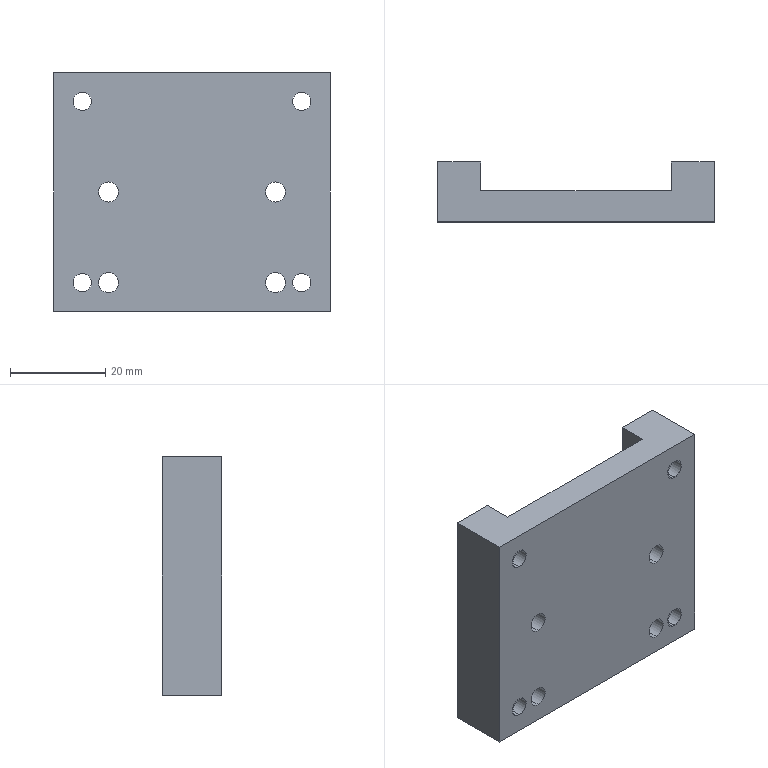Component | SolidWorks | PusherBlockSlideSeat-1 | 1 solid | 34 faces | box 58 x 12.5 x 50 mm | volume 23197 mm3 | cylinder 16 | plane 10 | cone 8 | commonest cylinder face diameters 4.2 x16
build123d program:
from build123d import *

# Parameters (mm, degrees)
SKETCH1_W             = 58
SKETCH1_H             = 50
BOSS_EXTRUDE1_DEPTH   = 12.5
SKETCH2_W             = 40
SKETCH2_H             = 78.188
CUT_EXTRUDE1_DEPTH    = 6
SKETCH6_W             = 20
SKETCH6_H             = 12.5
CUT_EXTRUDE2_DEPTH    = 12
BOSS_EXTRUDE2_DEPTH   = 12
M5_TAPPED_HOLE2_D     = 4.2
M5_TAPPED_HOLE2_DEPTH = 12.4
M5_TAPPED_HOLE2_TIP   = 1.262
M5_TAPPED_HOLE3_D     = 4.2
M5_TAPPED_HOLE3_DEPTH = 12.4
M5_TAPPED_HOLE3_TIP   = 1.262


with BuildPart() as part:
    # Sketch1 → Boss-Extrude1 (new body)
    with BuildSketch(Plane(origin=(0, 0, 0), x_dir=(1, 0, 0), z_dir=(0, 1, 0))):
        with Locations((-41.142, -16.579)):
            Rectangle(SKETCH1_W, SKETCH1_H)
    extrude(amount=BOSS_EXTRUDE1_DEPTH)

    # Sketch2 → Cut-Extrude1 (cut)
    with BuildSketch(Plane(origin=(0, 12.5, 0), x_dir=(1, 0, 0), z_dir=(0, 1, 0))):
        with Locations((-41.142, -23.387)):
            Rectangle(SKETCH2_W, SKETCH2_H)
    extrude(amount=-CUT_EXTRUDE1_DEPTH, mode=Mode.SUBTRACT)

    # Sketch6 → Cut-Extrude2 (cut)
    with BuildSketch(Plane.XY.offset(41.579)):
        with Locations((-22.142, 6.25)):
            Rectangle(SKETCH6_W, SKETCH6_H)
    extrude(amount=-CUT_EXTRUDE2_DEPTH, mode=Mode.SUBTRACT)

    # Sketch8 → Boss-Extrude2 (add)
    with BuildSketch(Plane.XY.offset(29.579)):
        Polygon((-32.142, 6.5), (-21.142, 6.5), (-21.142, 12.5), (-12.142, 12.5), (-12.142, 0), (-32.142, 0), align=None)
    extrude(amount=BOSS_EXTRUDE2_DEPTH)

    # M5 Tapped Hole2
    with Locations(Plane(origin=(0, 12.5, 0), x_dir=(-1, 0, 0), z_dir=(0, 1, 0))):
        with Locations((64.142, -2.421), (64.142, 35.579), (18.142, -2.421), (18.142, 35.579)):
            Hole(M5_TAPPED_HOLE2_D / 2, depth=M5_TAPPED_HOLE2_DEPTH)
            with Locations((0, 0, -(M5_TAPPED_HOLE2_DEPTH + M5_TAPPED_HOLE2_TIP / 2))):  # 118° drill point
                Cone(0, M5_TAPPED_HOLE2_D / 2, M5_TAPPED_HOLE2_TIP, mode=Mode.SUBTRACT)

    # M5 Tapped Hole3
    with Locations(Plane.XZ):
        with Locations((-23.642, -2.421), (-23.642, 16.579), (-58.642, 16.579), (-58.642, -2.421)):
            Hole(M5_TAPPED_HOLE3_D / 2, depth=M5_TAPPED_HOLE3_DEPTH)
            with Locations((0, 0, -(M5_TAPPED_HOLE3_DEPTH + M5_TAPPED_HOLE3_TIP / 2))):  # 118° drill point
                Cone(0, M5_TAPPED_HOLE3_D / 2, M5_TAPPED_HOLE3_TIP, mode=Mode.SUBTRACT)


solid = part.part

# Placed as in the assembly
solid = solid.moved(Location((34.227, -1.305, 60), (0, 0, 0)))
STEP:
#1=COLOUR_RGB('',0.7922,0.8196,0.9333);
#2=FILL_AREA_STYLE_COLOUR('',#1);
#3=FILL_AREA_STYLE('',(#2));
#4=SURFACE_STYLE_FILL_AREA(#3);
#5=SURFACE_SIDE_STYLE('',(#4));
#6=SURFACE_STYLE_USAGE(.BOTH.,#5);
#7=PRESENTATION_STYLE_ASSIGNMENT((#6));
#8=CARTESIAN_POINT('',(0.4167,0.2045,2.184));
#9=VERTEX_POINT('',#8);
#10=CARTESIAN_POINT('',(0.4167,0.2045,2.35));
#11=VERTEX_POINT('',#10);
#12=CARTESIAN_POINT('',(0.4167,0.2045,2.267));
#13=DIRECTION('',(0.,1.,0.));
#14=DIRECTION('',(0.,0.,1.));
#15=AXIS2_PLACEMENT_3D('',#12,#13,#14);
#16=CIRCLE('',#15,0.08268);
#17=EDGE_CURVE('',#9,#11,#16,.T.);
#18=ORIENTED_EDGE('',*,*,#17,.T.);
#19=CARTESIAN_POINT('',(0.4167,-0.05139,2.35));
#20=VERTEX_POINT('',#19);
#21=CARTESIAN_POINT('',(0.4167,-0.05139,2.35));
#22=DIRECTION('',(0.,-1.,0.));
#23=VECTOR('',#22,39.37);
#24=LINE('',#21,#23);
#25=EDGE_CURVE('',#11,#20,#24,.T.);
#26=ORIENTED_EDGE('',*,*,#25,.T.);
#27=CARTESIAN_POINT('',(0.4167,-0.05139,2.184));
#28=VERTEX_POINT('',#27);
#29=CARTESIAN_POINT('',(0.4167,-0.05139,2.267));
#30=DIRECTION('',(0.,-1.,0.));
#31=DIRECTION('',(0.,0.,-1.));
#32=AXIS2_PLACEMENT_3D('',#29,#30,#31);
#33=CIRCLE('',#32,0.08268);
#34=EDGE_CURVE('',#20,#28,#33,.T.);
#35=ORIENTED_EDGE('',*,*,#34,.T.);
#36=CARTESIAN_POINT('',(0.4167,-0.05139,2.184));
#37=DIRECTION('',(0.,-1.,0.));
#38=VECTOR('',#37,39.37);
#39=LINE('',#36,#38);
#40=EDGE_CURVE('',#9,#28,#39,.T.);
#41=ORIENTED_EDGE('',*,*,#40,.F.);
#42=EDGE_LOOP('',(#18,#26,#35,#41));
#43=FACE_OUTER_BOUND('',#42,.T.);
#44=CARTESIAN_POINT('',(0.4167,-0.05139,2.267));
#45=DIRECTION('',(0.,-1.,0.));
#46=DIRECTION('',(0.,0.,-1.));
#47=AXIS2_PLACEMENT_3D('',#44,#45,#46);
#48=CYLINDRICAL_SURFACE('',#47,0.08268);
#49=ADVANCED_FACE('',(#43),#48,.F.);
#50=CARTESIAN_POINT('',(0.4167,0.2045,2.932));
#51=VERTEX_POINT('',#50);
#52=CARTESIAN_POINT('',(0.4167,0.2045,3.098));
#53=VERTEX_POINT('',#52);
#54=CARTESIAN_POINT('',(0.4167,0.2045,3.015));
#55=DIRECTION('',(0.,1.,0.));
#56=DIRECTION('',(0.,0.,1.));
#57=AXIS2_PLACEMENT_3D('',#54,#55,#56);
#58=CIRCLE('',#57,0.08268);
#59=EDGE_CURVE('',#51,#53,#58,.T.);
#60=ORIENTED_EDGE('',*,*,#59,.T.);
#61=CARTESIAN_POINT('',(0.4167,-0.05139,3.098));
#62=VERTEX_POINT('',#61);
#63=CARTESIAN_POINT('',(0.4167,-0.05139,3.098));
#64=DIRECTION('',(0.,-1.,0.));
#65=VECTOR('',#64,39.37);
#66=LINE('',#63,#65);
#67=EDGE_CURVE('',#53,#62,#66,.T.);
#68=ORIENTED_EDGE('',*,*,#67,.T.);
#69=CARTESIAN_POINT('',(0.4167,-0.05139,2.932));
#70=VERTEX_POINT('',#69);
#71=CARTESIAN_POINT('',(0.4167,-0.05139,3.015));
#72=DIRECTION('',(0.,-1.,0.));
#73=DIRECTION('',(0.,0.,-1.));
#74=AXIS2_PLACEMENT_3D('',#71,#72,#73);
#75=CIRCLE('',#74,0.08268);
#76=EDGE_CURVE('',#62,#70,#75,.T.);
#77=ORIENTED_EDGE('',*,*,#76,.T.);
#78=CARTESIAN_POINT('',(0.4167,-0.05139,2.932));
#79=DIRECTION('',(0.,-1.,0.));
#80=VECTOR('',#79,39.37);
#81=LINE('',#78,#80);
#82=EDGE_CURVE('',#51,#70,#81,.T.);
#83=ORIENTED_EDGE('',*,*,#82,.F.);
#84=EDGE_LOOP('',(#60,#68,#77,#83));
#85=FACE_OUTER_BOUND('',#84,.T.);
#86=CARTESIAN_POINT('',(0.4167,-0.05139,3.015));
#87=DIRECTION('',(0.,-1.,0.));
#88=DIRECTION('',(0.,0.,-1.));
#89=AXIS2_PLACEMENT_3D('',#86,#87,#88);
#90=CYLINDRICAL_SURFACE('',#89,0.08268);
#91=ADVANCED_FACE('',(#85),#90,.F.);
#92=CARTESIAN_POINT('',(-0.9612,0.2045,2.932));
#93=VERTEX_POINT('',#92);
#94=CARTESIAN_POINT('',(-0.9612,0.2045,3.098));
#95=VERTEX_POINT('',#94);
#96=CARTESIAN_POINT('',(-0.9612,0.2045,3.015));
#97=DIRECTION('',(0.,1.,0.));
#98=DIRECTION('',(0.,0.,1.));
#99=AXIS2_PLACEMENT_3D('',#96,#97,#98);
#100=CIRCLE('',#99,0.08268);
#101=EDGE_CURVE('',#93,#95,#100,.T.);
#102=ORIENTED_EDGE('',*,*,#101,.T.);
#103=CARTESIAN_POINT('',(-0.9612,-0.05139,3.098));
#104=VERTEX_POINT('',#103);
#105=CARTESIAN_POINT('',(-0.9612,-0.05139,3.098));
#106=DIRECTION('',(0.,-1.,0.));
#107=VECTOR('',#106,39.37);
#108=LINE('',#105,#107);
#109=EDGE_CURVE('',#95,#104,#108,.T.);
#110=ORIENTED_EDGE('',*,*,#109,.T.);
#111=CARTESIAN_POINT('',(-0.9612,-0.05139,2.932));
#112=VERTEX_POINT('',#111);
#113=CARTESIAN_POINT('',(-0.9612,-0.05139,3.015));
#114=DIRECTION('',(0.,-1.,0.));
#115=DIRECTION('',(0.,0.,-1.));
#116=AXIS2_PLACEMENT_3D('',#113,#114,#115);
#117=CIRCLE('',#116,0.08268);
#118=EDGE_CURVE('',#104,#112,#117,.T.);
#119=ORIENTED_EDGE('',*,*,#118,.T.);
#120=CARTESIAN_POINT('',(-0.9612,-0.05139,2.932));
#121=DIRECTION('',(0.,-1.,0.));
#122=VECTOR('',#121,39.37);
#123=LINE('',#120,#122);
#124=EDGE_CURVE('',#93,#112,#123,.T.);
#125=ORIENTED_EDGE('',*,*,#124,.F.);
#126=EDGE_LOOP('',(#102,#110,#119,#125));
#127=FACE_OUTER_BOUND('',#126,.T.);
#128=CARTESIAN_POINT('',(-0.9612,-0.05139,3.015));
#129=DIRECTION('',(0.,-1.,0.));
#130=DIRECTION('',(0.,0.,-1.));
#131=AXIS2_PLACEMENT_3D('',#128,#129,#130);
#132=CYLINDRICAL_SURFACE('',#131,0.08268);
#133=ADVANCED_FACE('',(#127),#132,.F.);
#134=CARTESIAN_POINT('',(-0.9612,0.2045,2.184));
#135=VERTEX_POINT('',#134);
#136=CARTESIAN_POINT('',(-0.9612,0.2045,2.35));
#137=VERTEX_POINT('',#136);
#138=CARTESIAN_POINT('',(-0.9612,0.2045,2.267));
#139=DIRECTION('',(0.,1.,0.));
#140=DIRECTION('',(0.,0.,1.));
#141=AXIS2_PLACEMENT_3D('',#138,#139,#140);
#142=CIRCLE('',#141,0.08268);
#143=EDGE_CURVE('',#135,#137,#142,.T.);
#144=ORIENTED_EDGE('',*,*,#143,.T.);
#145=CARTESIAN_POINT('',(-0.9612,-0.05139,2.35));
#146=VERTEX_POINT('',#145);
#147=CARTESIAN_POINT('',(-0.9612,-0.05139,2.35));
#148=DIRECTION('',(0.,-1.,0.));
#149=VECTOR('',#148,39.37);
#150=LINE('',#147,#149);
#151=EDGE_CURVE('',#137,#146,#150,.T.);
#152=ORIENTED_EDGE('',*,*,#151,.T.);
#153=CARTESIAN_POINT('',(-0.9612,-0.05139,2.184));
#154=VERTEX_POINT('',#153);
#155=CARTESIAN_POINT('',(-0.9612,-0.05139,2.267));
#156=DIRECTION('',(0.,-1.,0.));
#157=DIRECTION('',(0.,0.,-1.));
#158=AXIS2_PLACEMENT_3D('',#155,#156,#157);
#159=CIRCLE('',#158,0.08268);
#160=EDGE_CURVE('',#146,#154,#159,.T.);
#161=ORIENTED_EDGE('',*,*,#160,.T.);
#162=CARTESIAN_POINT('',(-0.9612,-0.05139,2.184));
#163=DIRECTION('',(0.,-1.,0.));
#164=VECTOR('',#163,39.37);
#165=LINE('',#162,#164);
#166=EDGE_CURVE('',#135,#154,#165,.T.);
#167=ORIENTED_EDGE('',*,*,#166,.F.);
#168=EDGE_LOOP('',(#144,#152,#161,#167));
#169=FACE_OUTER_BOUND('',#168,.T.);
#170=CARTESIAN_POINT('',(-0.9612,-0.05139,2.267));
#171=DIRECTION('',(0.,-1.,0.));
#172=DIRECTION('',(0.,0.,-1.));
#173=AXIS2_PLACEMENT_3D('',#170,#171,#172);
#174=CYLINDRICAL_SURFACE('',#173,0.08268);
#175=ADVANCED_FACE('',(#169),#174,.F.);
#176=CARTESIAN_POINT('',(-1.178,-0.04745,2.184));
#177=VERTEX_POINT('',#176);
#178=CARTESIAN_POINT('',(-1.178,-0.04745,2.35));
#179=VERTEX_POINT('',#178);
#180=CARTESIAN_POINT('',(-1.178,-0.04745,2.267));
#181=DIRECTION('',(0.,1.,0.));
#182=DIRECTION('',(0.,0.,1.));
#183=AXIS2_PLACEMENT_3D('',#180,#181,#182);
#184=CIRCLE('',#183,0.08268);
#185=EDGE_CURVE('',#177,#179,#184,.T.);
#186=ORIENTED_EDGE('',*,*,#185,.F.);
#187=CARTESIAN_POINT('',(-1.178,0.4407,2.184));
#188=VERTEX_POINT('',#187);
#189=CARTESIAN_POINT('',(-1.178,0.4407,2.184));
#190=DIRECTION('',(0.,1.,0.));
#191=VECTOR('',#190,39.37);
#192=LINE('',#189,#191);
#193=EDGE_CURVE('',#177,#188,#192,.T.);
#194=ORIENTED_EDGE('',*,*,#193,.T.);
#195=CARTESIAN_POINT('',(-1.178,0.4407,2.35));
#196=VERTEX_POINT('',#195);
#197=CARTESIAN_POINT('',(-1.178,0.4407,2.267));
#198=DIRECTION('',(0.,1.,0.));
#199=DIRECTION('',(0.,0.,1.));
#200=AXIS2_PLACEMENT_3D('',#197,#198,#199);
#201=CIRCLE('',#200,0.08268);
#202=EDGE_CURVE('',#188,#196,#201,.T.);
#203=ORIENTED_EDGE('',*,*,#202,.T.);
#204=CARTESIAN_POINT('',(-1.178,0.4407,2.35));
#205=DIRECTION('',(0.,1.,0.));
#206=VECTOR('',#205,39.37);
#207=LINE('',#204,#206);
#208=EDGE_CURVE('',#179,#196,#207,.T.);
#209=ORIENTED_EDGE('',*,*,#208,.F.);
#210=EDGE_LOOP('',(#186,#194,#203,#209));
#211=FACE_OUTER_BOUND('',#210,.T.);
#212=CARTESIAN_POINT('',(-1.178,0.4407,2.267));
#213=DIRECTION('',(0.,1.,0.));
#214=DIRECTION('',(0.,0.,1.));
#215=AXIS2_PLACEMENT_3D('',#212,#213,#214);
#216=CYLINDRICAL_SURFACE('',#215,0.08268);
#217=ADVANCED_FACE('',(#211),#216,.F.);
#218=CARTESIAN_POINT('',(-1.178,-0.05139,2.191));
#219=VERTEX_POINT('',#218);
#220=CARTESIAN_POINT('',(-1.178,-0.05139,2.343));
#221=VERTEX_POINT('',#220);
#222=CARTESIAN_POINT('',(-1.178,-0.05139,2.267));
#223=DIRECTION('',(0.,1.,0.));
#224=DIRECTION('',(0.,0.,1.));
#225=AXIS2_PLACEMENT_3D('',#222,#223,#224);
#226=CIRCLE('',#225,0.07612);
#227=EDGE_CURVE('',#219,#221,#226,.T.);
#228=ORIENTED_EDGE('',*,*,#227,.F.);
#229=CARTESIAN_POINT('',(-1.178,-0.04745,2.184));
#230=DIRECTION('',(0.,0.515,-0.8572));
#231=VECTOR('',#230,39.37);
#232=LINE('',#229,#231);
#233=EDGE_CURVE('',#219,#177,#232,.T.);
#234=ORIENTED_EDGE('',*,*,#233,.T.);
#235=ORIENTED_EDGE('',*,*,#185,.T.);
#236=CARTESIAN_POINT('',(-1.178,-0.04745,2.35));
#237=DIRECTION('',(0.,0.515,0.8572));
#238=VECTOR('',#237,39.37);
#239=LINE('',#236,#238);
#240=EDGE_CURVE('',#221,#179,#239,.T.);
#241=ORIENTED_EDGE('',*,*,#240,.F.);
#242=EDGE_LOOP('',(#228,#234,#235,#241));
#243=FACE_OUTER_BOUND('',#242,.T.);
#244=CARTESIAN_POINT('',(-1.178,-0.04745,2.267));
#245=DIRECTION('',(0.,1.,0.));
#246=DIRECTION('',(0.,0.,1.));
#247=AXIS2_PLACEMENT_3D('',#244,#245,#246);
#248=CONICAL_SURFACE('',#247,0.08268,1.03);
#249=ADVANCED_FACE('',(#243),#248,.F.);
#250=CARTESIAN_POINT('',(-1.178,-0.04745,3.68));
#251=VERTEX_POINT('',#250);
#252=CARTESIAN_POINT('',(-1.178,-0.04745,3.846));
#253=VERTEX_POINT('',#252);
#254=CARTESIAN_POINT('',(-1.178,-0.04745,3.763));
#255=DIRECTION('',(0.,1.,0.));
#256=DIRECTION('',(0.,0.,1.));
#257=AXIS2_PLACEMENT_3D('',#254,#255,#256);
#258=CIRCLE('',#257,0.08268);
#259=EDGE_CURVE('',#251,#253,#258,.T.);
#260=ORIENTED_EDGE('',*,*,#259,.F.);
#261=CARTESIAN_POINT('',(-1.178,0.4407,3.68));
#262=VERTEX_POINT('',#261);
#263=CARTESIAN_POINT('',(-1.178,0.4407,3.68));
#264=DIRECTION('',(0.,1.,0.));
#265=VECTOR('',#264,39.37);
#266=LINE('',#263,#265);
#267=EDGE_CURVE('',#251,#262,#266,.T.);
#268=ORIENTED_EDGE('',*,*,#267,.T.);
#269=CARTESIAN_POINT('',(-1.178,0.4407,3.846));
#270=VERTEX_POINT('',#269);
#271=CARTESIAN_POINT('',(-1.178,0.4407,3.763));
#272=DIRECTION('',(0.,1.,0.));
#273=DIRECTION('',(0.,0.,1.));
#274=AXIS2_PLACEMENT_3D('',#271,#272,#273);
#275=CIRCLE('',#274,0.08268);
#276=EDGE_CURVE('',#262,#270,#275,.T.);
#277=ORIENTED_EDGE('',*,*,#276,.T.);
#278=CARTESIAN_POINT('',(-1.178,0.4407,3.846));
#279=DIRECTION('',(0.,1.,0.));
#280=VECTOR('',#279,39.37);
#281=LINE('',#278,#280);
#282=EDGE_CURVE('',#253,#270,#281,.T.);
#283=ORIENTED_EDGE('',*,*,#282,.F.);
#284=EDGE_LOOP('',(#260,#268,#277,#283));
#285=FACE_OUTER_BOUND('',#284,.T.);
#286=CARTESIAN_POINT('',(-1.178,0.4407,3.763));
#287=DIRECTION('',(0.,1.,0.));
#288=DIRECTION('',(0.,0.,1.));
#289=AXIS2_PLACEMENT_3D('',#286,#287,#288);
#290=CYLINDRICAL_SURFACE('',#289,0.08268);
#291=ADVANCED_FACE('',(#285),#290,.F.);
#292=CARTESIAN_POINT('',(-1.178,-0.05139,3.687));
#293=VERTEX_POINT('',#292);
#294=CARTESIAN_POINT('',(-1.178,-0.05139,3.839));
#295=VERTEX_POINT('',#294);
#296=CARTESIAN_POINT('',(-1.178,-0.05139,3.763));
#297=DIRECTION('',(0.,1.,0.));
#298=DIRECTION('',(0.,0.,1.));
#299=AXIS2_PLACEMENT_3D('',#296,#297,#298);
#300=CIRCLE('',#299,0.07612);
#301=EDGE_CURVE('',#293,#295,#300,.T.);
#302=ORIENTED_EDGE('',*,*,#301,.F.);
#303=CARTESIAN_POINT('',(-1.178,-0.04745,3.68));
#304=DIRECTION('',(0.,0.515,-0.8572));
#305=VECTOR('',#304,39.37);
#306=LINE('',#303,#305);
#307=EDGE_CURVE('',#293,#251,#306,.T.);
#308=ORIENTED_EDGE('',*,*,#307,.T.);
#309=ORIENTED_EDGE('',*,*,#259,.T.);
#310=CARTESIAN_POINT('',(-1.178,-0.04745,3.846));
#311=DIRECTION('',(0.,0.515,0.8572));
#312=VECTOR('',#311,39.37);
#313=LINE('',#310,#312);
#314=EDGE_CURVE('',#295,#253,#313,.T.);
#315=ORIENTED_EDGE('',*,*,#314,.F.);
#316=EDGE_LOOP('',(#302,#308,#309,#315));
#317=FACE_OUTER_BOUND('',#316,.T.);
#318=CARTESIAN_POINT('',(-1.178,-0.04745,3.763));
#319=DIRECTION('',(0.,1.,0.));
#320=DIRECTION('',(0.,0.,1.));
#321=AXIS2_PLACEMENT_3D('',#318,#319,#320);
#322=CONICAL_SURFACE('',#321,0.08268,1.03);
#323=ADVANCED_FACE('',(#317),#322,.F.);
#324=CARTESIAN_POINT('',(0.6333,-0.04745,2.184));
#325=VERTEX_POINT('',#324);
#326=CARTESIAN_POINT('',(0.6333,-0.04745,2.35));
#327=VERTEX_POINT('',#326);
#328=CARTESIAN_POINT('',(0.6333,-0.04745,2.267));
#329=DIRECTION('',(0.,1.,0.));
#330=DIRECTION('',(0.,0.,1.));
#331=AXIS2_PLACEMENT_3D('',#328,#329,#330);
#332=CIRCLE('',#331,0.08268);
#333=EDGE_CURVE('',#325,#327,#332,.T.);
#334=ORIENTED_EDGE('',*,*,#333,.F.);
#335=CARTESIAN_POINT('',(0.6333,0.4407,2.184));
#336=VERTEX_POINT('',#335);
#337=CARTESIAN_POINT('',(0.6333,0.4407,2.184));
#338=DIRECTION('',(0.,1.,0.));
#339=VECTOR('',#338,39.37);
#340=LINE('',#337,#339);
#341=EDGE_CURVE('',#325,#336,#340,.T.);
#342=ORIENTED_EDGE('',*,*,#341,.T.);
#343=CARTESIAN_POINT('',(0.6333,0.4407,2.35));
#344=VERTEX_POINT('',#343);
#345=CARTESIAN_POINT('',(0.6333,0.4407,2.267));
#346=DIRECTION('',(0.,1.,0.));
#347=DIRECTION('',(0.,0.,1.));
#348=AXIS2_PLACEMENT_3D('',#345,#346,#347);
#349=CIRCLE('',#348,0.08268);
#350=EDGE_CURVE('',#336,#344,#349,.T.);
#351=ORIENTED_EDGE('',*,*,#350,.T.);
#352=CARTESIAN_POINT('',(0.6333,0.4407,2.35));
#353=DIRECTION('',(0.,1.,0.));
#354=VECTOR('',#353,39.37);
#355=LINE('',#352,#354);
#356=EDGE_CURVE('',#327,#344,#355,.T.);
#357=ORIENTED_EDGE('',*,*,#356,.F.);
#358=EDGE_LOOP('',(#334,#342,#351,#357));
#359=FACE_OUTER_BOUND('',#358,.T.);
#360=CARTESIAN_POINT('',(0.6333,0.4407,2.267));
#361=DIRECTION('',(0.,1.,0.));
#362=DIRECTION('',(0.,0.,1.));
#363=AXIS2_PLACEMENT_3D('',#360,#361,#362);
#364=CYLINDRICAL_SURFACE('',#363,0.08268);
#365=ADVANCED_FACE('',(#359),#364,.F.);
#366=CARTESIAN_POINT('',(0.6333,-0.05139,2.191));
#367=VERTEX_POINT('',#366);
#368=CARTESIAN_POINT('',(0.6333,-0.05139,2.343));
#369=VERTEX_POINT('',#368);
#370=CARTESIAN_POINT('',(0.6333,-0.05139,2.267));
#371=DIRECTION('',(0.,1.,0.));
#372=DIRECTION('',(0.,0.,1.));
#373=AXIS2_PLACEMENT_3D('',#370,#371,#372);
#374=CIRCLE('',#373,0.07612);
#375=EDGE_CURVE('',#367,#369,#374,.T.);
#376=ORIENTED_EDGE('',*,*,#375,.F.);
#377=CARTESIAN_POINT('',(0.6333,-0.04745,2.184));
#378=DIRECTION('',(0.,0.515,-0.8572));
#379=VECTOR('',#378,39.37);
#380=LINE('',#377,#379);
#381=EDGE_CURVE('',#367,#325,#380,.T.);
#382=ORIENTED_EDGE('',*,*,#381,.T.);
#383=ORIENTED_EDGE('',*,*,#333,.T.);
#384=CARTESIAN_POINT('',(0.6333,-0.04745,2.35));
#385=DIRECTION('',(0.,0.515,0.8572));
#386=VECTOR('',#385,39.37);
#387=LINE('',#384,#386);
#388=EDGE_CURVE('',#369,#327,#387,.T.);
#389=ORIENTED_EDGE('',*,*,#388,.F.);
#390=EDGE_LOOP('',(#376,#382,#383,#389));
#391=FACE_OUTER_BOUND('',#390,.T.);
#392=CARTESIAN_POINT('',(0.6333,-0.04745,2.267));
#393=DIRECTION('',(0.,1.,0.));
#394=DIRECTION('',(0.,0.,1.));
#395=AXIS2_PLACEMENT_3D('',#392,#393,#394);
#396=CONICAL_SURFACE('',#395,0.08268,1.03);
#397=ADVANCED_FACE('',(#391),#396,.F.);
#398=CARTESIAN_POINT('',(0.6333,-0.04745,3.68));
#399=VERTEX_POINT('',#398);
#400=CARTESIAN_POINT('',(0.6333,-0.04745,3.846));
#401=VERTEX_POINT('',#400);
#402=CARTESIAN_POINT('',(0.6333,-0.04745,3.763));
#403=DIRECTION('',(0.,1.,0.));
#404=DIRECTION('',(0.,0.,1.));
#405=AXIS2_PLACEMENT_3D('',#402,#403,#404);
#406=CIRCLE('',#405,0.08268);
#407=EDGE_CURVE('',#399,#401,#406,.T.);
#408=ORIENTED_EDGE('',*,*,#407,.F.);
#409=CARTESIAN_POINT('',(0.6333,0.4407,3.68));
#410=VERTEX_POINT('',#409);
#411=CARTESIAN_POINT('',(0.6333,0.4407,3.68));
#412=DIRECTION('',(0.,1.,0.));
#413=VECTOR('',#412,39.37);
#414=LINE('',#411,#413);
#415=EDGE_CURVE('',#399,#410,#414,.T.);
#416=ORIENTED_EDGE('',*,*,#415,.T.);
#417=CARTESIAN_POINT('',(0.6333,0.4407,3.846));
#418=VERTEX_POINT('',#417);
#419=CARTESIAN_POINT('',(0.6333,0.4407,3.763));
#420=DIRECTION('',(0.,1.,0.));
#421=DIRECTION('',(0.,0.,1.));
#422=AXIS2_PLACEMENT_3D('',#419,#420,#421);
#423=CIRCLE('',#422,0.08268);
#424=EDGE_CURVE('',#410,#418,#423,.T.);
#425=ORIENTED_EDGE('',*,*,#424,.T.);
#426=CARTESIAN_POINT('',(0.6333,0.4407,3.846));
#427=DIRECTION('',(0.,1.,0.));
#428=VECTOR('',#427,39.37);
#429=LINE('',#426,#428);
#430=EDGE_CURVE('',#401,#418,#429,.T.);
#431=ORIENTED_EDGE('',*,*,#430,.F.);
#432=EDGE_LOOP('',(#408,#416,#425,#431));
#433=FACE_OUTER_BOUND('',#432,.T.);
#434=CARTESIAN_POINT('',(0.6333,0.4407,3.763));
#435=DIRECTION('',(0.,1.,0.));
#436=DIRECTION('',(0.,0.,1.));
#437=AXIS2_PLACEMENT_3D('',#434,#435,#436);
#438=CYLINDRICAL_SURFACE('',#437,0.08268);
#439=ADVANCED_FACE('',(#433),#438,.F.);
#440=CARTESIAN_POINT('',(0.6333,-0.05139,3.687));
#441=VERTEX_POINT('',#440);
#442=CARTESIAN_POINT('',(0.6333,-0.05139,3.839));
#443=VERTEX_POINT('',#442);
#444=CARTESIAN_POINT('',(0.6333,-0.05139,3.763));
#445=DIRECTION('',(0.,1.,0.));
#446=DIRECTION('',(0.,0.,1.));
#447=AXIS2_PLACEMENT_3D('',#444,#445,#446);
#448=CIRCLE('',#447,0.07612);
#449=EDGE_CURVE('',#441,#443,#448,.T.);
#450=ORIENTED_EDGE('',*,*,#449,.F.);
#451=CARTESIAN_POINT('',(0.6333,-0.04745,3.68));
#452=DIRECTION('',(0.,0.515,-0.8572));
#453=VECTOR('',#452,39.37);
#454=LINE('',#451,#453);
#455=EDGE_CURVE('',#441,#399,#454,.T.);
#456=ORIENTED_EDGE('',*,*,#455,.T.);
#457=ORIENTED_EDGE('',*,*,#407,.T.);
#458=CARTESIAN_POINT('',(0.6333,-0.04745,3.846));
#459=DIRECTION('',(0.,0.515,0.8572));
#460=VECTOR('',#459,39.37);
#461=LINE('',#458,#460);
#462=EDGE_CURVE('',#443,#401,#461,.T.);
#463=ORIENTED_EDGE('',*,*,#462,.F.);
#464=EDGE_LOOP('',(#450,#456,#457,#463));
#465=FACE_OUTER_BOUND('',#464,.T.);
#466=CARTESIAN_POINT('',(0.6333,-0.04745,3.763));
#467=DIRECTION('',(0.,1.,0.));
#468=DIRECTION('',(0.,0.,1.));
#469=AXIS2_PLACEMENT_3D('',#466,#467,#468);
#470=CONICAL_SURFACE('',#469,0.08268,1.03);
#471=ADVANCED_FACE('',(#465),#470,.F.);
#472=CARTESIAN_POINT('',(0.8695,0.4407,3.999));
#473=VERTEX_POINT('',#472);
#474=CARTESIAN_POINT('',(0.8695,0.4407,2.031));
#475=VERTEX_POINT('',#474);
#476=CARTESIAN_POINT('',(0.8695,0.4407,2.031));
#477=DIRECTION('',(-0.,0.,-1.));
#478=VECTOR('',#477,39.37);
#479=LINE('',#476,#478);
#480=EDGE_CURVE('',#473,#475,#479,.T.);
#481=ORIENTED_EDGE('',*,*,#480,.F.);
#482=CARTESIAN_POINT('',(0.8695,-0.05139,3.999));
#483=VERTEX_POINT('',#482);
#484=CARTESIAN_POINT('',(0.8695,0.4407,3.999));
#485=DIRECTION('',(0.,-1.,0.));
#486=VECTOR('',#485,39.37);
#487=LINE('',#484,#486);
#488=EDGE_CURVE('',#473,#483,#487,.T.);
#489=ORIENTED_EDGE('',*,*,#488,.T.);
#490=CARTESIAN_POINT('',(0.8695,-0.05139,2.031));
#491=VERTEX_POINT('',#490);
#492=CARTESIAN_POINT('',(0.8695,-0.05139,2.031));
#493=DIRECTION('',(-0.,0.,-1.));
#494=VECTOR('',#493,39.37);
#495=LINE('',#492,#494);
#496=EDGE_CURVE('',#483,#491,#495,.T.);
#497=ORIENTED_EDGE('',*,*,#496,.T.);
#498=CARTESIAN_POINT('',(0.8695,0.4407,2.031));
#499=DIRECTION('',(0.,-1.,0.));
#500=VECTOR('',#499,39.37);
#501=LINE('',#498,#500);
#502=EDGE_CURVE('',#475,#491,#501,.T.);
#503=ORIENTED_EDGE('',*,*,#502,.F.);
#504=EDGE_LOOP('',(#481,#489,#497,#503));
#505=FACE_OUTER_BOUND('',#504,.T.);
#506=CARTESIAN_POINT('',(0.8695,0.4407,2.031));
#507=DIRECTION('',(-1.,0.,0.));
#508=DIRECTION('',(0.,0.,1.));
#509=AXIS2_PLACEMENT_3D('',#506,#507,#508);
#510=PLANE('',#509);
#511=ADVANCED_FACE('',(#505),#510,.F.);
#512=CARTESIAN_POINT('',(0.6333,0.4407,2.267));
#513=DIRECTION('',(0.,1.,0.));
#514=DIRECTION('',(0.,0.,1.));
#515=AXIS2_PLACEMENT_3D('',#512,#513,#514);
#516=CIRCLE('',#515,0.08268);
#517=EDGE_CURVE('',#344,#336,#516,.T.);
#518=ORIENTED_EDGE('',*,*,#517,.F.);
#519=ORIENTED_EDGE('',*,*,#350,.F.);
#520=EDGE_LOOP('',(#518,#519));
#521=FACE_BOUND('',#520,.T.);
#522=CARTESIAN_POINT('',(0.6333,0.4407,3.763));
#523=DIRECTION('',(0.,1.,0.));
#524=DIRECTION('',(0.,0.,1.));
#525=AXIS2_PLACEMENT_3D('',#522,#523,#524);
#526=CIRCLE('',#525,0.08268);
#527=EDGE_CURVE('',#418,#410,#526,.T.);
#528=ORIENTED_EDGE('',*,*,#527,.F.);
#529=ORIENTED_EDGE('',*,*,#424,.F.);
#530=EDGE_LOOP('',(#528,#529));
#531=FACE_BOUND('',#530,.T.);
#532=CARTESIAN_POINT('',(0.5152,0.4407,3.999));
#533=VERTEX_POINT('',#532);
#534=CARTESIAN_POINT('',(0.5152,0.4407,2.031));
#535=VERTEX_POINT('',#534);
#536=CARTESIAN_POINT('',(0.5152,0.4407,3.999));
#537=DIRECTION('',(-0.,0.,-1.));
#538=VECTOR('',#537,39.37);
#539=LINE('',#536,#538);
#540=EDGE_CURVE('',#533,#535,#539,.T.);
#541=ORIENTED_EDGE('',*,*,#540,.F.);
#542=CARTESIAN_POINT('',(0.5152,0.4407,3.999));
#543=DIRECTION('',(1.,0.,0.));
#544=VECTOR('',#543,39.37);
#545=LINE('',#542,#544);
#546=EDGE_CURVE('',#533,#473,#545,.T.);
#547=ORIENTED_EDGE('',*,*,#546,.T.);
#548=ORIENTED_EDGE('',*,*,#480,.T.);
#549=CARTESIAN_POINT('',(-1.414,0.4407,2.031));
#550=DIRECTION('',(-1.,0.,0.));
#551=VECTOR('',#550,39.37);
#552=LINE('',#549,#551);
#553=EDGE_CURVE('',#475,#535,#552,.T.);
#554=ORIENTED_EDGE('',*,*,#553,.T.);
#555=EDGE_LOOP('',(#541,#547,#548,#554));
#556=FACE_OUTER_BOUND('',#555,.T.);
#557=CARTESIAN_POINT('',(-1.414,0.4407,3.999));
#558=DIRECTION('',(0.,1.,0.));
#559=DIRECTION('',(0.,0.,1.));
#560=AXIS2_PLACEMENT_3D('',#557,#558,#559);
#561=PLANE('',#560);
#562=ADVANCED_FACE('',(#521,#531,#556),#561,.T.);
#563=CARTESIAN_POINT('',(0.5152,0.2045,3.999));
#564=VERTEX_POINT('',#563);
#565=CARTESIAN_POINT('',(0.5152,0.2045,2.031));
#566=VERTEX_POINT('',#565);
#567=CARTESIAN_POINT('',(0.5152,0.2045,1.744));
#568=DIRECTION('',(-0.,0.,-1.));
#569=VECTOR('',#568,39.37);
#570=LINE('',#567,#569);
#571=EDGE_CURVE('',#564,#566,#570,.T.);
#572=ORIENTED_EDGE('',*,*,#571,.F.);
#573=CARTESIAN_POINT('',(0.5152,0.2045,3.999));
#574=DIRECTION('',(0.,1.,0.));
#575=VECTOR('',#574,39.37);
#576=LINE('',#573,#575);
#577=EDGE_CURVE('',#564,#533,#576,.T.);
#578=ORIENTED_EDGE('',*,*,#577,.T.);
#579=ORIENTED_EDGE('',*,*,#540,.T.);
#580=CARTESIAN_POINT('',(0.5152,0.4407,2.031));
#581=DIRECTION('',(0.,1.,0.));
#582=VECTOR('',#581,39.37);
#583=LINE('',#580,#582);
#584=EDGE_CURVE('',#566,#535,#583,.T.);
#585=ORIENTED_EDGE('',*,*,#584,.F.);
#586=EDGE_LOOP('',(#572,#578,#579,#585));
#587=FACE_OUTER_BOUND('',#586,.T.);
#588=CARTESIAN_POINT('',(0.5152,0.2045,1.744));
#589=DIRECTION('',(1.,0.,-0.));
#590=DIRECTION('',(-0.,0.,-1.));
#591=AXIS2_PLACEMENT_3D('',#588,#589,#590);
#592=PLANE('',#591);
#593=ADVANCED_FACE('',(#587),#592,.F.);
#594=CARTESIAN_POINT('',(-1.178,0.4407,2.267));
#595=DIRECTION('',(0.,1.,0.));
#596=DIRECTION('',(0.,0.,1.));
#597=AXIS2_PLACEMENT_3D('',#594,#595,#596);
#598=CIRCLE('',#597,0.08268);
#599=EDGE_CURVE('',#196,#188,#598,.T.);
#600=ORIENTED_EDGE('',*,*,#599,.F.);
#601=ORIENTED_EDGE('',*,*,#202,.F.);
#602=EDGE_LOOP('',(#600,#601));
#603=FACE_BOUND('',#602,.T.);
#604=CARTESIAN_POINT('',(-1.178,0.4407,3.763));
#605=DIRECTION('',(0.,1.,0.));
#606=DIRECTION('',(0.,0.,1.));
#607=AXIS2_PLACEMENT_3D('',#604,#605,#606);
#608=CIRCLE('',#607,0.08268);
#609=EDGE_CURVE('',#270,#262,#608,.T.);
#610=ORIENTED_EDGE('',*,*,#609,.F.);
#611=ORIENTED_EDGE('',*,*,#276,.F.);
#612=EDGE_LOOP('',(#610,#611));
#613=FACE_BOUND('',#612,.T.);
#614=CARTESIAN_POINT('',(-1.06,0.4407,2.031));
#615=VERTEX_POINT('',#614);
#616=CARTESIAN_POINT('',(-1.06,0.4407,3.999));
#617=VERTEX_POINT('',#616);
#618=CARTESIAN_POINT('',(-1.06,0.4407,3.999));
#619=DIRECTION('',(0.,0.,1.));
#620=VECTOR('',#619,39.37);
#621=LINE('',#618,#620);
#622=EDGE_CURVE('',#615,#617,#621,.T.);
#623=ORIENTED_EDGE('',*,*,#622,.F.);
#624=CARTESIAN_POINT('',(-1.414,0.4407,2.031));
#625=VERTEX_POINT('',#624);
#626=CARTESIAN_POINT('',(-1.414,0.4407,2.031));
#627=DIRECTION('',(-1.,0.,0.));
#628=VECTOR('',#627,39.37);
#629=LINE('',#626,#628);
#630=EDGE_CURVE('',#615,#625,#629,.T.);
#631=ORIENTED_EDGE('',*,*,#630,.T.);
#632=CARTESIAN_POINT('',(-1.414,0.4407,3.999));
#633=VERTEX_POINT('',#632);
#634=CARTESIAN_POINT('',(-1.414,0.4407,2.031));
#635=DIRECTION('',(0.,0.,1.));
#636=VECTOR('',#635,39.37);
#637=LINE('',#634,#636);
#638=EDGE_CURVE('',#625,#633,#637,.T.);
#639=ORIENTED_EDGE('',*,*,#638,.T.);
#640=CARTESIAN_POINT('',(-1.414,0.4407,3.999));
#641=DIRECTION('',(1.,0.,0.));
#642=VECTOR('',#641,39.37);
#643=LINE('',#640,#642);
#644=EDGE_CURVE('',#633,#617,#643,.T.);
#645=ORIENTED_EDGE('',*,*,#644,.T.);
#646=EDGE_LOOP('',(#623,#631,#639,#645));
#647=FACE_OUTER_BOUND('',#646,.T.);
#648=CARTESIAN_POINT('',(-1.414,0.4407,3.999));
#649=DIRECTION('',(0.,1.,0.));
#650=DIRECTION('',(0.,0.,1.));
#651=AXIS2_PLACEMENT_3D('',#648,#649,#650);
#652=PLANE('',#651);
#653=ADVANCED_FACE('',(#603,#613,#647),#652,.T.);
#654=CARTESIAN_POINT('',(-1.414,-0.05139,2.031));
#655=VERTEX_POINT('',#654);
#656=CARTESIAN_POINT('',(-1.414,-0.05139,3.999));
#657=VERTEX_POINT('',#656);
#658=CARTESIAN_POINT('',(-1.414,-0.05139,2.031));
#659=DIRECTION('',(0.,0.,1.));
#660=VECTOR('',#659,39.37);
#661=LINE('',#658,#660);
#662=EDGE_CURVE('',#655,#657,#661,.T.);
#663=ORIENTED_EDGE('',*,*,#662,.T.);
#664=CARTESIAN_POINT('',(-1.414,0.4407,3.999));
#665=DIRECTION('',(0.,-1.,0.));
#666=VECTOR('',#665,39.37);
#667=LINE('',#664,#666);
#668=EDGE_CURVE('',#633,#657,#667,.T.);
#669=ORIENTED_EDGE('',*,*,#668,.F.);
#670=ORIENTED_EDGE('',*,*,#638,.F.);
#671=CARTESIAN_POINT('',(-1.414,0.4407,2.031));
#672=DIRECTION('',(0.,-1.,0.));
#673=VECTOR('',#672,39.37);
#674=LINE('',#671,#673);
#675=EDGE_CURVE('',#625,#655,#674,.T.);
#676=ORIENTED_EDGE('',*,*,#675,.T.);
#677=EDGE_LOOP('',(#663,#669,#670,#676));
#678=FACE_OUTER_BOUND('',#677,.T.);
#679=CARTESIAN_POINT('',(-1.414,0.4407,2.031));
#680=DIRECTION('',(1.,0.,0.));
#681=DIRECTION('',(0.,0.,-1.));
#682=AXIS2_PLACEMENT_3D('',#679,#680,#681);
#683=PLANE('',#682);
#684=ADVANCED_FACE('',(#678),#683,.F.);
#685=CARTESIAN_POINT('',(-1.414,-0.05139,3.999));
#686=DIRECTION('',(1.,0.,0.));
#687=VECTOR('',#686,39.37);
#688=LINE('',#685,#687);
#689=EDGE_CURVE('',#657,#483,#688,.T.);
#690=ORIENTED_EDGE('',*,*,#689,.T.);
#691=ORIENTED_EDGE('',*,*,#488,.F.);
#692=ORIENTED_EDGE('',*,*,#546,.F.);
#693=ORIENTED_EDGE('',*,*,#577,.F.);
#694=CARTESIAN_POINT('',(-1.06,0.2045,3.999));
#695=VERTEX_POINT('',#694);
#696=CARTESIAN_POINT('',(-1.414,0.2045,3.999));
#697=DIRECTION('',(1.,0.,0.));
#698=VECTOR('',#697,39.37);
#699=LINE('',#696,#698);
#700=EDGE_CURVE('',#695,#564,#699,.T.);
#701=ORIENTED_EDGE('',*,*,#700,.F.);
#702=CARTESIAN_POINT('',(-1.06,0.4407,3.999));
#703=DIRECTION('',(0.,1.,0.));
#704=VECTOR('',#703,39.37);
#705=LINE('',#702,#704);
#706=EDGE_CURVE('',#695,#617,#705,.T.);
#707=ORIENTED_EDGE('',*,*,#706,.T.);
#708=ORIENTED_EDGE('',*,*,#644,.F.);
#709=ORIENTED_EDGE('',*,*,#668,.T.);
#710=EDGE_LOOP('',(#690,#691,#692,#693,#701,#707,#708,#709));
#711=FACE_OUTER_BOUND('',#710,.T.);
#712=CARTESIAN_POINT('',(-1.414,0.4407,3.999));
#713=DIRECTION('',(0.,0.,-1.));
#714=DIRECTION('',(-1.,0.,0.));
#715=AXIS2_PLACEMENT_3D('',#712,#713,#714);
#716=PLANE('',#715);
#717=ADVANCED_FACE('',(#711),#716,.F.);
#718=ORIENTED_EDGE('',*,*,#630,.F.);
#719=CARTESIAN_POINT('',(-1.06,0.2045,2.031));
#720=VERTEX_POINT('',#719);
#721=CARTESIAN_POINT('',(-1.06,0.4407,2.031));
#722=DIRECTION('',(0.,-1.,0.));
#723=VECTOR('',#722,39.37);
#724=LINE('',#721,#723);
#725=EDGE_CURVE('',#615,#720,#724,.T.);
#726=ORIENTED_EDGE('',*,*,#725,.T.);
#727=CARTESIAN_POINT('',(-1.414,0.2045,2.031));
#728=DIRECTION('',(-1.,0.,0.));
#729=VECTOR('',#728,39.37);
#730=LINE('',#727,#729);
#731=EDGE_CURVE('',#566,#720,#730,.T.);
#732=ORIENTED_EDGE('',*,*,#731,.F.);
#733=ORIENTED_EDGE('',*,*,#584,.T.);
#734=ORIENTED_EDGE('',*,*,#553,.F.);
#735=ORIENTED_EDGE('',*,*,#502,.T.);
#736=CARTESIAN_POINT('',(-1.414,-0.05139,2.031));
#737=DIRECTION('',(-1.,0.,0.));
#738=VECTOR('',#737,39.37);
#739=LINE('',#736,#738);
#740=EDGE_CURVE('',#491,#655,#739,.T.);
#741=ORIENTED_EDGE('',*,*,#740,.T.);
#742=ORIENTED_EDGE('',*,*,#675,.F.);
#743=EDGE_LOOP('',(#718,#726,#732,#733,#734,#735,#741,#742));
#744=FACE_OUTER_BOUND('',#743,.T.);
#745=CARTESIAN_POINT('',(-1.414,0.4407,2.031));
#746=DIRECTION('',(0.,0.,1.));
#747=DIRECTION('',(1.,0.,0.));
#748=AXIS2_PLACEMENT_3D('',#745,#746,#747);
#749=PLANE('',#748);
#750=ADVANCED_FACE('',(#744),#749,.F.);
#751=CARTESIAN_POINT('',(0.4167,-0.05139,2.267));
#752=DIRECTION('',(0.,-1.,0.));
#753=DIRECTION('',(0.,0.,-1.));
#754=AXIS2_PLACEMENT_3D('',#751,#752,#753);
#755=CIRCLE('',#754,0.08268);
#756=EDGE_CURVE('',#28,#20,#755,.T.);
#757=ORIENTED_EDGE('',*,*,#756,.F.);
#758=ORIENTED_EDGE('',*,*,#34,.F.);
#759=EDGE_LOOP('',(#757,#758));
#760=FACE_BOUND('',#759,.T.);
#761=CARTESIAN_POINT('',(0.4167,-0.05139,3.015));
#762=DIRECTION('',(0.,-1.,0.));
#763=DIRECTION('',(0.,0.,-1.));
#764=AXIS2_PLACEMENT_3D('',#761,#762,#763);
#765=CIRCLE('',#764,0.08268);
#766=EDGE_CURVE('',#70,#62,#765,.T.);
#767=ORIENTED_EDGE('',*,*,#766,.F.);
#768=ORIENTED_EDGE('',*,*,#76,.F.);
#769=EDGE_LOOP('',(#767,#768));
#770=FACE_BOUND('',#769,.T.);
#771=CARTESIAN_POINT('',(-0.9612,-0.05139,3.015));
#772=DIRECTION('',(0.,-1.,0.));
#773=DIRECTION('',(0.,0.,-1.));
#774=AXIS2_PLACEMENT_3D('',#771,#772,#773);
#775=CIRCLE('',#774,0.08268);
#776=EDGE_CURVE('',#112,#104,#775,.T.);
#777=ORIENTED_EDGE('',*,*,#776,.F.);
#778=ORIENTED_EDGE('',*,*,#118,.F.);
#779=EDGE_LOOP('',(#777,#778));
#780=FACE_BOUND('',#779,.T.);
#781=CARTESIAN_POINT('',(-0.9612,-0.05139,2.267));
#782=DIRECTION('',(0.,-1.,0.));
#783=DIRECTION('',(0.,0.,-1.));
#784=AXIS2_PLACEMENT_3D('',#781,#782,#783);
#785=CIRCLE('',#784,0.08268);
#786=EDGE_CURVE('',#154,#146,#785,.T.);
#787=ORIENTED_EDGE('',*,*,#786,.F.);
#788=ORIENTED_EDGE('',*,*,#160,.F.);
#789=EDGE_LOOP('',(#787,#788));
#790=FACE_BOUND('',#789,.T.);
#791=CARTESIAN_POINT('',(-1.178,-0.05139,2.267));
#792=DIRECTION('',(0.,1.,0.));
#793=DIRECTION('',(0.,0.,1.));
#794=AXIS2_PLACEMENT_3D('',#791,#792,#793);
#795=CIRCLE('',#794,0.07612);
#796=EDGE_CURVE('',#221,#219,#795,.T.);
#797=ORIENTED_EDGE('',*,*,#796,.T.);
#798=ORIENTED_EDGE('',*,*,#227,.T.);
#799=EDGE_LOOP('',(#797,#798));
#800=FACE_BOUND('',#799,.T.);
#801=CARTESIAN_POINT('',(-1.178,-0.05139,3.763));
#802=DIRECTION('',(0.,1.,0.));
#803=DIRECTION('',(0.,0.,1.));
#804=AXIS2_PLACEMENT_3D('',#801,#802,#803);
#805=CIRCLE('',#804,0.07612);
#806=EDGE_CURVE('',#295,#293,#805,.T.);
#807=ORIENTED_EDGE('',*,*,#806,.T.);
#808=ORIENTED_EDGE('',*,*,#301,.T.);
#809=EDGE_LOOP('',(#807,#808));
#810=FACE_BOUND('',#809,.T.);
#811=CARTESIAN_POINT('',(0.6333,-0.05139,2.267));
#812=DIRECTION('',(0.,1.,0.));
#813=DIRECTION('',(0.,0.,1.));
#814=AXIS2_PLACEMENT_3D('',#811,#812,#813);
#815=CIRCLE('',#814,0.07612);
#816=EDGE_CURVE('',#369,#367,#815,.T.);
#817=ORIENTED_EDGE('',*,*,#816,.T.);
#818=ORIENTED_EDGE('',*,*,#375,.T.);
#819=EDGE_LOOP('',(#817,#818));
#820=FACE_BOUND('',#819,.T.);
#821=CARTESIAN_POINT('',(0.6333,-0.05139,3.763));
#822=DIRECTION('',(0.,1.,0.));
#823=DIRECTION('',(0.,0.,1.));
#824=AXIS2_PLACEMENT_3D('',#821,#822,#823);
#825=CIRCLE('',#824,0.07612);
#826=EDGE_CURVE('',#443,#441,#825,.T.);
#827=ORIENTED_EDGE('',*,*,#826,.T.);
#828=ORIENTED_EDGE('',*,*,#449,.T.);
#829=EDGE_LOOP('',(#827,#828));
#830=FACE_BOUND('',#829,.T.);
#831=ORIENTED_EDGE('',*,*,#496,.F.);
#832=ORIENTED_EDGE('',*,*,#689,.F.);
#833=ORIENTED_EDGE('',*,*,#662,.F.);
#834=ORIENTED_EDGE('',*,*,#740,.F.);
#835=EDGE_LOOP('',(#831,#832,#833,#834));
#836=FACE_OUTER_BOUND('',#835,.T.);
#837=CARTESIAN_POINT('',(-1.414,-0.05139,3.999));
#838=DIRECTION('',(0.,1.,0.));
#839=DIRECTION('',(0.,0.,1.));
#840=AXIS2_PLACEMENT_3D('',#837,#838,#839);
#841=PLANE('',#840);
#842=ADVANCED_FACE('',(#760,#770,#780,#790,#800,#810,#820,#830,#836),#841,.F.);
#843=ORIENTED_EDGE('',*,*,#17,.F.);
#844=CARTESIAN_POINT('',(0.4167,0.2045,2.267));
#845=DIRECTION('',(0.,1.,0.));
#846=DIRECTION('',(0.,0.,1.));
#847=AXIS2_PLACEMENT_3D('',#844,#845,#846);
#848=CIRCLE('',#847,0.08268);
#849=EDGE_CURVE('',#11,#9,#848,.T.);
#850=ORIENTED_EDGE('',*,*,#849,.F.);
#851=EDGE_LOOP('',(#843,#850));
#852=FACE_BOUND('',#851,.T.);
#853=ORIENTED_EDGE('',*,*,#59,.F.);
#854=CARTESIAN_POINT('',(0.4167,0.2045,3.015));
#855=DIRECTION('',(0.,1.,0.));
#856=DIRECTION('',(0.,0.,1.));
#857=AXIS2_PLACEMENT_3D('',#854,#855,#856);
#858=CIRCLE('',#857,0.08268);
#859=EDGE_CURVE('',#53,#51,#858,.T.);
#860=ORIENTED_EDGE('',*,*,#859,.F.);
#861=EDGE_LOOP('',(#853,#860));
#862=FACE_BOUND('',#861,.T.);
#863=ORIENTED_EDGE('',*,*,#101,.F.);
#864=CARTESIAN_POINT('',(-0.9612,0.2045,3.015));
#865=DIRECTION('',(0.,1.,0.));
#866=DIRECTION('',(0.,0.,1.));
#867=AXIS2_PLACEMENT_3D('',#864,#865,#866);
#868=CIRCLE('',#867,0.08268);
#869=EDGE_CURVE('',#95,#93,#868,.T.);
#870=ORIENTED_EDGE('',*,*,#869,.F.);
#871=EDGE_LOOP('',(#863,#870));
#872=FACE_BOUND('',#871,.T.);
#873=ORIENTED_EDGE('',*,*,#143,.F.);
#874=CARTESIAN_POINT('',(-0.9612,0.2045,2.267));
#875=DIRECTION('',(0.,1.,0.));
#876=DIRECTION('',(0.,0.,1.));
#877=AXIS2_PLACEMENT_3D('',#874,#875,#876);
#878=CIRCLE('',#877,0.08268);
#879=EDGE_CURVE('',#137,#135,#878,.T.);
#880=ORIENTED_EDGE('',*,*,#879,.F.);
#881=EDGE_LOOP('',(#873,#880));
#882=FACE_BOUND('',#881,.T.);
#883=ORIENTED_EDGE('',*,*,#700,.T.);
#884=ORIENTED_EDGE('',*,*,#571,.T.);
#885=ORIENTED_EDGE('',*,*,#731,.T.);
#886=CARTESIAN_POINT('',(-1.06,0.2045,1.744));
#887=DIRECTION('',(0.,0.,1.));
#888=VECTOR('',#887,39.37);
#889=LINE('',#886,#888);
#890=EDGE_CURVE('',#720,#695,#889,.T.);
#891=ORIENTED_EDGE('',*,*,#890,.T.);
#892=EDGE_LOOP('',(#883,#884,#885,#891));
#893=FACE_OUTER_BOUND('',#892,.T.);
#894=CARTESIAN_POINT('',(-1.06,0.2045,4.822));
#895=DIRECTION('',(0.,1.,0.));
#896=DIRECTION('',(0.,0.,1.));
#897=AXIS2_PLACEMENT_3D('',#894,#895,#896);
#898=PLANE('',#897);
#899=ADVANCED_FACE('',(#852,#862,#872,#882,#893),#898,.T.);
#900=ORIENTED_EDGE('',*,*,#890,.F.);
#901=ORIENTED_EDGE('',*,*,#725,.F.);
#902=ORIENTED_EDGE('',*,*,#622,.T.);
#903=ORIENTED_EDGE('',*,*,#706,.F.);
#904=EDGE_LOOP('',(#900,#901,#902,#903));
#905=FACE_OUTER_BOUND('',#904,.T.);
#906=CARTESIAN_POINT('',(-1.06,0.2045,1.744));
#907=DIRECTION('',(-1.,0.,0.));
#908=DIRECTION('',(0.,0.,1.));
#909=AXIS2_PLACEMENT_3D('',#906,#907,#908);
#910=PLANE('',#909);
#911=ADVANCED_FACE('',(#905),#910,.F.);
#912=ORIENTED_EDGE('',*,*,#455,.F.);
#913=ORIENTED_EDGE('',*,*,#826,.F.);
#914=ORIENTED_EDGE('',*,*,#462,.T.);
#915=CARTESIAN_POINT('',(0.6333,-0.04745,3.763));
#916=DIRECTION('',(0.,1.,0.));
#917=DIRECTION('',(0.,0.,1.));
#918=AXIS2_PLACEMENT_3D('',#915,#916,#917);
#919=CIRCLE('',#918,0.08268);
#920=EDGE_CURVE('',#401,#399,#919,.T.);
#921=ORIENTED_EDGE('',*,*,#920,.T.);
#922=EDGE_LOOP('',(#912,#913,#914,#921));
#923=FACE_OUTER_BOUND('',#922,.T.);
#924=CARTESIAN_POINT('',(0.6333,-0.04745,3.763));
#925=DIRECTION('',(0.,1.,0.));
#926=DIRECTION('',(0.,0.,1.));
#927=AXIS2_PLACEMENT_3D('',#924,#925,#926);
#928=CONICAL_SURFACE('',#927,0.08268,1.03);
#929=ADVANCED_FACE('',(#923),#928,.F.);
#930=ORIENTED_EDGE('',*,*,#415,.F.);
#931=ORIENTED_EDGE('',*,*,#920,.F.);
#932=ORIENTED_EDGE('',*,*,#430,.T.);
#933=ORIENTED_EDGE('',*,*,#527,.T.);
#934=EDGE_LOOP('',(#930,#931,#932,#933));
#935=FACE_OUTER_BOUND('',#934,.T.);
#936=CARTESIAN_POINT('',(0.6333,0.4407,3.763));
#937=DIRECTION('',(0.,1.,0.));
#938=DIRECTION('',(0.,0.,1.));
#939=AXIS2_PLACEMENT_3D('',#936,#937,#938);
#940=CYLINDRICAL_SURFACE('',#939,0.08268);
#941=ADVANCED_FACE('',(#935),#940,.F.);
#942=ORIENTED_EDGE('',*,*,#381,.F.);
#943=ORIENTED_EDGE('',*,*,#816,.F.);
#944=ORIENTED_EDGE('',*,*,#388,.T.);
#945=CARTESIAN_POINT('',(0.6333,-0.04745,2.267));
#946=DIRECTION('',(0.,1.,0.));
#947=DIRECTION('',(0.,0.,1.));
#948=AXIS2_PLACEMENT_3D('',#945,#946,#947);
#949=CIRCLE('',#948,0.08268);
#950=EDGE_CURVE('',#327,#325,#949,.T.);
#951=ORIENTED_EDGE('',*,*,#950,.T.);
#952=EDGE_LOOP('',(#942,#943,#944,#951));
#953=FACE_OUTER_BOUND('',#952,.T.);
#954=CARTESIAN_POINT('',(0.6333,-0.04745,2.267));
#955=DIRECTION('',(0.,1.,0.));
#956=DIRECTION('',(0.,0.,1.));
#957=AXIS2_PLACEMENT_3D('',#954,#955,#956);
#958=CONICAL_SURFACE('',#957,0.08268,1.03);
#959=ADVANCED_FACE('',(#953),#958,.F.);
#960=ORIENTED_EDGE('',*,*,#341,.F.);
#961=ORIENTED_EDGE('',*,*,#950,.F.);
#962=ORIENTED_EDGE('',*,*,#356,.T.);
#963=ORIENTED_EDGE('',*,*,#517,.T.);
#964=EDGE_LOOP('',(#960,#961,#962,#963));
#965=FACE_OUTER_BOUND('',#964,.T.);
#966=CARTESIAN_POINT('',(0.6333,0.4407,2.267));
#967=DIRECTION('',(0.,1.,0.));
#968=DIRECTION('',(0.,0.,1.));
#969=AXIS2_PLACEMENT_3D('',#966,#967,#968);
#970=CYLINDRICAL_SURFACE('',#969,0.08268);
#971=ADVANCED_FACE('',(#965),#970,.F.);
#972=ORIENTED_EDGE('',*,*,#307,.F.);
#973=ORIENTED_EDGE('',*,*,#806,.F.);
#974=ORIENTED_EDGE('',*,*,#314,.T.);
#975=CARTESIAN_POINT('',(-1.178,-0.04745,3.763));
#976=DIRECTION('',(0.,1.,0.));
#977=DIRECTION('',(0.,0.,1.));
#978=AXIS2_PLACEMENT_3D('',#975,#976,#977);
#979=CIRCLE('',#978,0.08268);
#980=EDGE_CURVE('',#253,#251,#979,.T.);
#981=ORIENTED_EDGE('',*,*,#980,.T.);
#982=EDGE_LOOP('',(#972,#973,#974,#981));
#983=FACE_OUTER_BOUND('',#982,.T.);
#984=CARTESIAN_POINT('',(-1.178,-0.04745,3.763));
#985=DIRECTION('',(0.,1.,0.));
#986=DIRECTION('',(0.,0.,1.));
#987=AXIS2_PLACEMENT_3D('',#984,#985,#986);
#988=CONICAL_SURFACE('',#987,0.08268,1.03);
#989=ADVANCED_FACE('',(#983),#988,.F.);
#990=ORIENTED_EDGE('',*,*,#267,.F.);
#991=ORIENTED_EDGE('',*,*,#980,.F.);
#992=ORIENTED_EDGE('',*,*,#282,.T.);
#993=ORIENTED_EDGE('',*,*,#609,.T.);
#994=EDGE_LOOP('',(#990,#991,#992,#993));
#995=FACE_OUTER_BOUND('',#994,.T.);
#996=CARTESIAN_POINT('',(-1.178,0.4407,3.763));
#997=DIRECTION('',(0.,1.,0.));
#998=DIRECTION('',(0.,0.,1.));
#999=AXIS2_PLACEMENT_3D('',#996,#997,#998);
#1000=CYLINDRICAL_SURFACE('',#999,0.08268);
#1001=ADVANCED_FACE('',(#995),#1000,.F.);
#1002=ORIENTED_EDGE('',*,*,#233,.F.);
#1003=ORIENTED_EDGE('',*,*,#796,.F.);
#1004=ORIENTED_EDGE('',*,*,#240,.T.);
#1005=CARTESIAN_POINT('',(-1.178,-0.04745,2.267));
#1006=DIRECTION('',(0.,1.,0.));
#1007=DIRECTION('',(0.,0.,1.));
#1008=AXIS2_PLACEMENT_3D('',#1005,#1006,#1007);
#1009=CIRCLE('',#1008,0.08268);
#1010=EDGE_CURVE('',#179,#177,#1009,.T.);
#1011=ORIENTED_EDGE('',*,*,#1010,.T.);
#1012=EDGE_LOOP('',(#1002,#1003,#1004,#1011));
#1013=FACE_OUTER_BOUND('',#1012,.T.);
#1014=CARTESIAN_POINT('',(-1.178,-0.04745,2.267));
#1015=DIRECTION('',(0.,1.,0.));
#1016=DIRECTION('',(0.,0.,1.));
#1017=AXIS2_PLACEMENT_3D('',#1014,#1015,#1016);
#1018=CONICAL_SURFACE('',#1017,0.08268,1.03);
#1019=ADVANCED_FACE('',(#1013),#1018,.F.);
#1020=ORIENTED_EDGE('',*,*,#193,.F.);
#1021=ORIENTED_EDGE('',*,*,#1010,.F.);
#1022=ORIENTED_EDGE('',*,*,#208,.T.);
#1023=ORIENTED_EDGE('',*,*,#599,.T.);
#1024=EDGE_LOOP('',(#1020,#1021,#1022,#1023));
#1025=FACE_OUTER_BOUND('',#1024,.T.);
#1026=CARTESIAN_POINT('',(-1.178,0.4407,2.267));
#1027=DIRECTION('',(0.,1.,0.));
#1028=DIRECTION('',(0.,0.,1.));
#1029=AXIS2_PLACEMENT_3D('',#1026,#1027,#1028);
#1030=CYLINDRICAL_SURFACE('',#1029,0.08268);
#1031=ADVANCED_FACE('',(#1025),#1030,.F.);
#1032=ORIENTED_EDGE('',*,*,#151,.F.);
#1033=ORIENTED_EDGE('',*,*,#879,.T.);
#1034=ORIENTED_EDGE('',*,*,#166,.T.);
#1035=ORIENTED_EDGE('',*,*,#786,.T.);
#1036=EDGE_LOOP('',(#1032,#1033,#1034,#1035));
#1037=FACE_OUTER_BOUND('',#1036,.T.);
#1038=CARTESIAN_POINT('',(-0.9612,-0.05139,2.267));
#1039=DIRECTION('',(0.,-1.,0.));
#1040=DIRECTION('',(0.,0.,-1.));
#1041=AXIS2_PLACEMENT_3D('',#1038,#1039,#1040);
#1042=CYLINDRICAL_SURFACE('',#1041,0.08268);
#1043=ADVANCED_FACE('',(#1037),#1042,.F.);
#1044=ORIENTED_EDGE('',*,*,#109,.F.);
#1045=ORIENTED_EDGE('',*,*,#869,.T.);
#1046=ORIENTED_EDGE('',*,*,#124,.T.);
#1047=ORIENTED_EDGE('',*,*,#776,.T.);
#1048=EDGE_LOOP('',(#1044,#1045,#1046,#1047));
#1049=FACE_OUTER_BOUND('',#1048,.T.);
#1050=CARTESIAN_POINT('',(-0.9612,-0.05139,3.015));
#1051=DIRECTION('',(0.,-1.,0.));
#1052=DIRECTION('',(0.,0.,-1.));
#1053=AXIS2_PLACEMENT_3D('',#1050,#1051,#1052);
#1054=CYLINDRICAL_SURFACE('',#1053,0.08268);
#1055=ADVANCED_FACE('',(#1049),#1054,.F.);
#1056=ORIENTED_EDGE('',*,*,#67,.F.);
#1057=ORIENTED_EDGE('',*,*,#859,.T.);
#1058=ORIENTED_EDGE('',*,*,#82,.T.);
#1059=ORIENTED_EDGE('',*,*,#766,.T.);
#1060=EDGE_LOOP('',(#1056,#1057,#1058,#1059));
#1061=FACE_OUTER_BOUND('',#1060,.T.);
#1062=CARTESIAN_POINT('',(0.4167,-0.05139,3.015));
#1063=DIRECTION('',(0.,-1.,0.));
#1064=DIRECTION('',(0.,0.,-1.));
#1065=AXIS2_PLACEMENT_3D('',#1062,#1063,#1064);
#1066=CYLINDRICAL_SURFACE('',#1065,0.08268);
#1067=ADVANCED_FACE('',(#1061),#1066,.F.);
#1068=ORIENTED_EDGE('',*,*,#25,.F.);
#1069=ORIENTED_EDGE('',*,*,#849,.T.);
#1070=ORIENTED_EDGE('',*,*,#40,.T.);
#1071=ORIENTED_EDGE('',*,*,#756,.T.);
#1072=EDGE_LOOP('',(#1068,#1069,#1070,#1071));
#1073=FACE_OUTER_BOUND('',#1072,.T.);
#1074=CARTESIAN_POINT('',(0.4167,-0.05139,2.267));
#1075=DIRECTION('',(0.,-1.,0.));
#1076=DIRECTION('',(0.,0.,-1.));
#1077=AXIS2_PLACEMENT_3D('',#1074,#1075,#1076);
#1078=CYLINDRICAL_SURFACE('',#1077,0.08268);
#1079=ADVANCED_FACE('',(#1073),#1078,.F.);
#1080=CLOSED_SHELL('',(#49,#91,#133,#175,#217,#249,#291,#323,#365,#397,#439,#471,#511,#562,#593,#653,#684,#717,#750,#842,#899,#911,#929,#941,#959,#971,#989,#1001,#1019,#1031,#1043,#1055,#1067,#1079));
#1081=MANIFOLD_SOLID_BREP('',#1080);
#1082=STYLED_ITEM('',(#7),#1081);
#1083=PRESENTATION_LAYER_ASSIGNMENT('','',(#1082));
#1084=CARTESIAN_POINT('',(0.,0.,0.));
#1085=DIRECTION('',(0.,0.,1.));
#1086=DIRECTION('',(1.,0.,0.));
#1087=AXIS2_PLACEMENT_3D('',#1084,#1085,#1086);
#1088=(LENGTH_UNIT()NAMED_UNIT(*)SI_UNIT($,.METRE.));
#1089=LENGTH_MEASURE_WITH_UNIT(LENGTH_MEASURE(0.0254),#1088);
#1090=DIMENSIONAL_EXPONENTS(1.,0.,0.,0.,0.,0.,0.);
#1091=(CONVERSION_BASED_UNIT('',#1089)LENGTH_UNIT()NAMED_UNIT(#1090));
#1092=UNCERTAINTY_MEASURE_WITH_UNIT(LENGTH_MEASURE(0.00001),#1091,'','');
#1093=(NAMED_UNIT(*)PLANE_ANGLE_UNIT()SI_UNIT($,.RADIAN.));
#1094=(NAMED_UNIT(*)SI_UNIT($,.STERADIAN.)SOLID_ANGLE_UNIT());
#1095=(GEOMETRIC_REPRESENTATION_CONTEXT(3)GLOBAL_UNCERTAINTY_ASSIGNED_CONTEXT((#1092))GLOBAL_UNIT_ASSIGNED_CONTEXT((#1091,#1093,#1094))REPRESENTATION_CONTEXT('',''));
#1096=ADVANCED_BREP_SHAPE_REPRESENTATION('',(#1081,#1087),#1095);
#1097=(LENGTH_UNIT()NAMED_UNIT(*)SI_UNIT($,.METRE.));
#1098=LENGTH_MEASURE_WITH_UNIT(LENGTH_MEASURE(0.0254),#1097);
#1099=DIMENSIONAL_EXPONENTS(1.,0.,0.,0.,0.,0.,0.);
#1100=(CONVERSION_BASED_UNIT('',#1098)LENGTH_UNIT()NAMED_UNIT(#1099));
#1101=UNCERTAINTY_MEASURE_WITH_UNIT(LENGTH_MEASURE(0.00001),#1100,'','');
#1102=(NAMED_UNIT(*)PLANE_ANGLE_UNIT()SI_UNIT($,.RADIAN.));
#1103=(NAMED_UNIT(*)SI_UNIT($,.STERADIAN.)SOLID_ANGLE_UNIT());
#1104=(GEOMETRIC_REPRESENTATION_CONTEXT(3)GLOBAL_UNCERTAINTY_ASSIGNED_CONTEXT((#1101))GLOBAL_UNIT_ASSIGNED_CONTEXT((#1100,#1102,#1103))REPRESENTATION_CONTEXT('',''));
#1105=MECHANICAL_DESIGN_GEOMETRIC_PRESENTATION_REPRESENTATION('',(#1082),#1104);